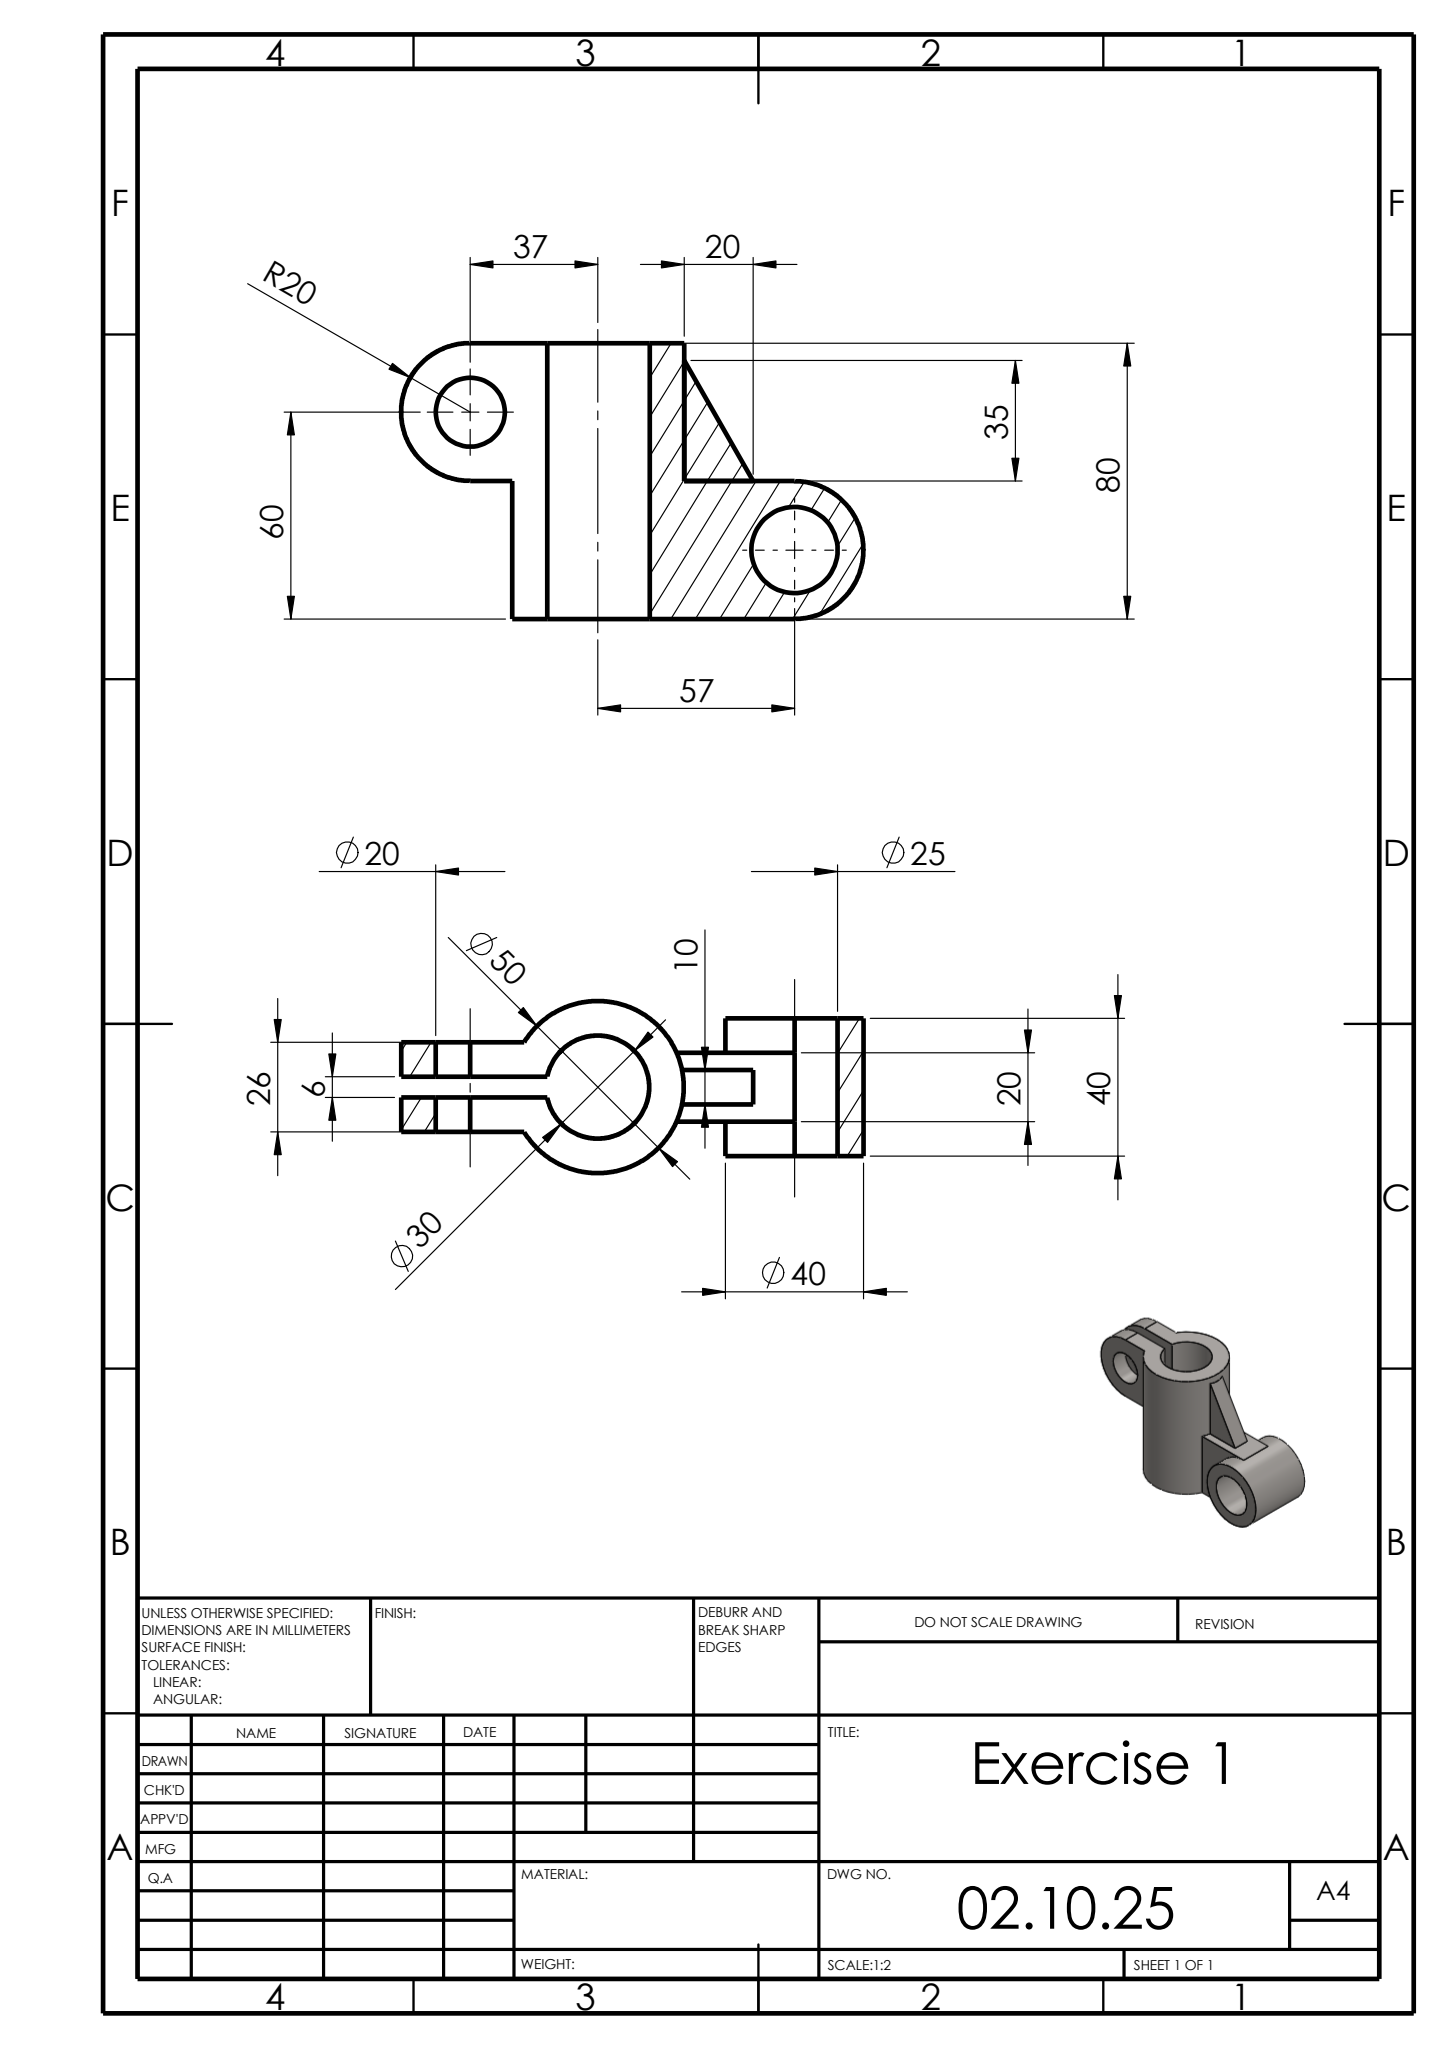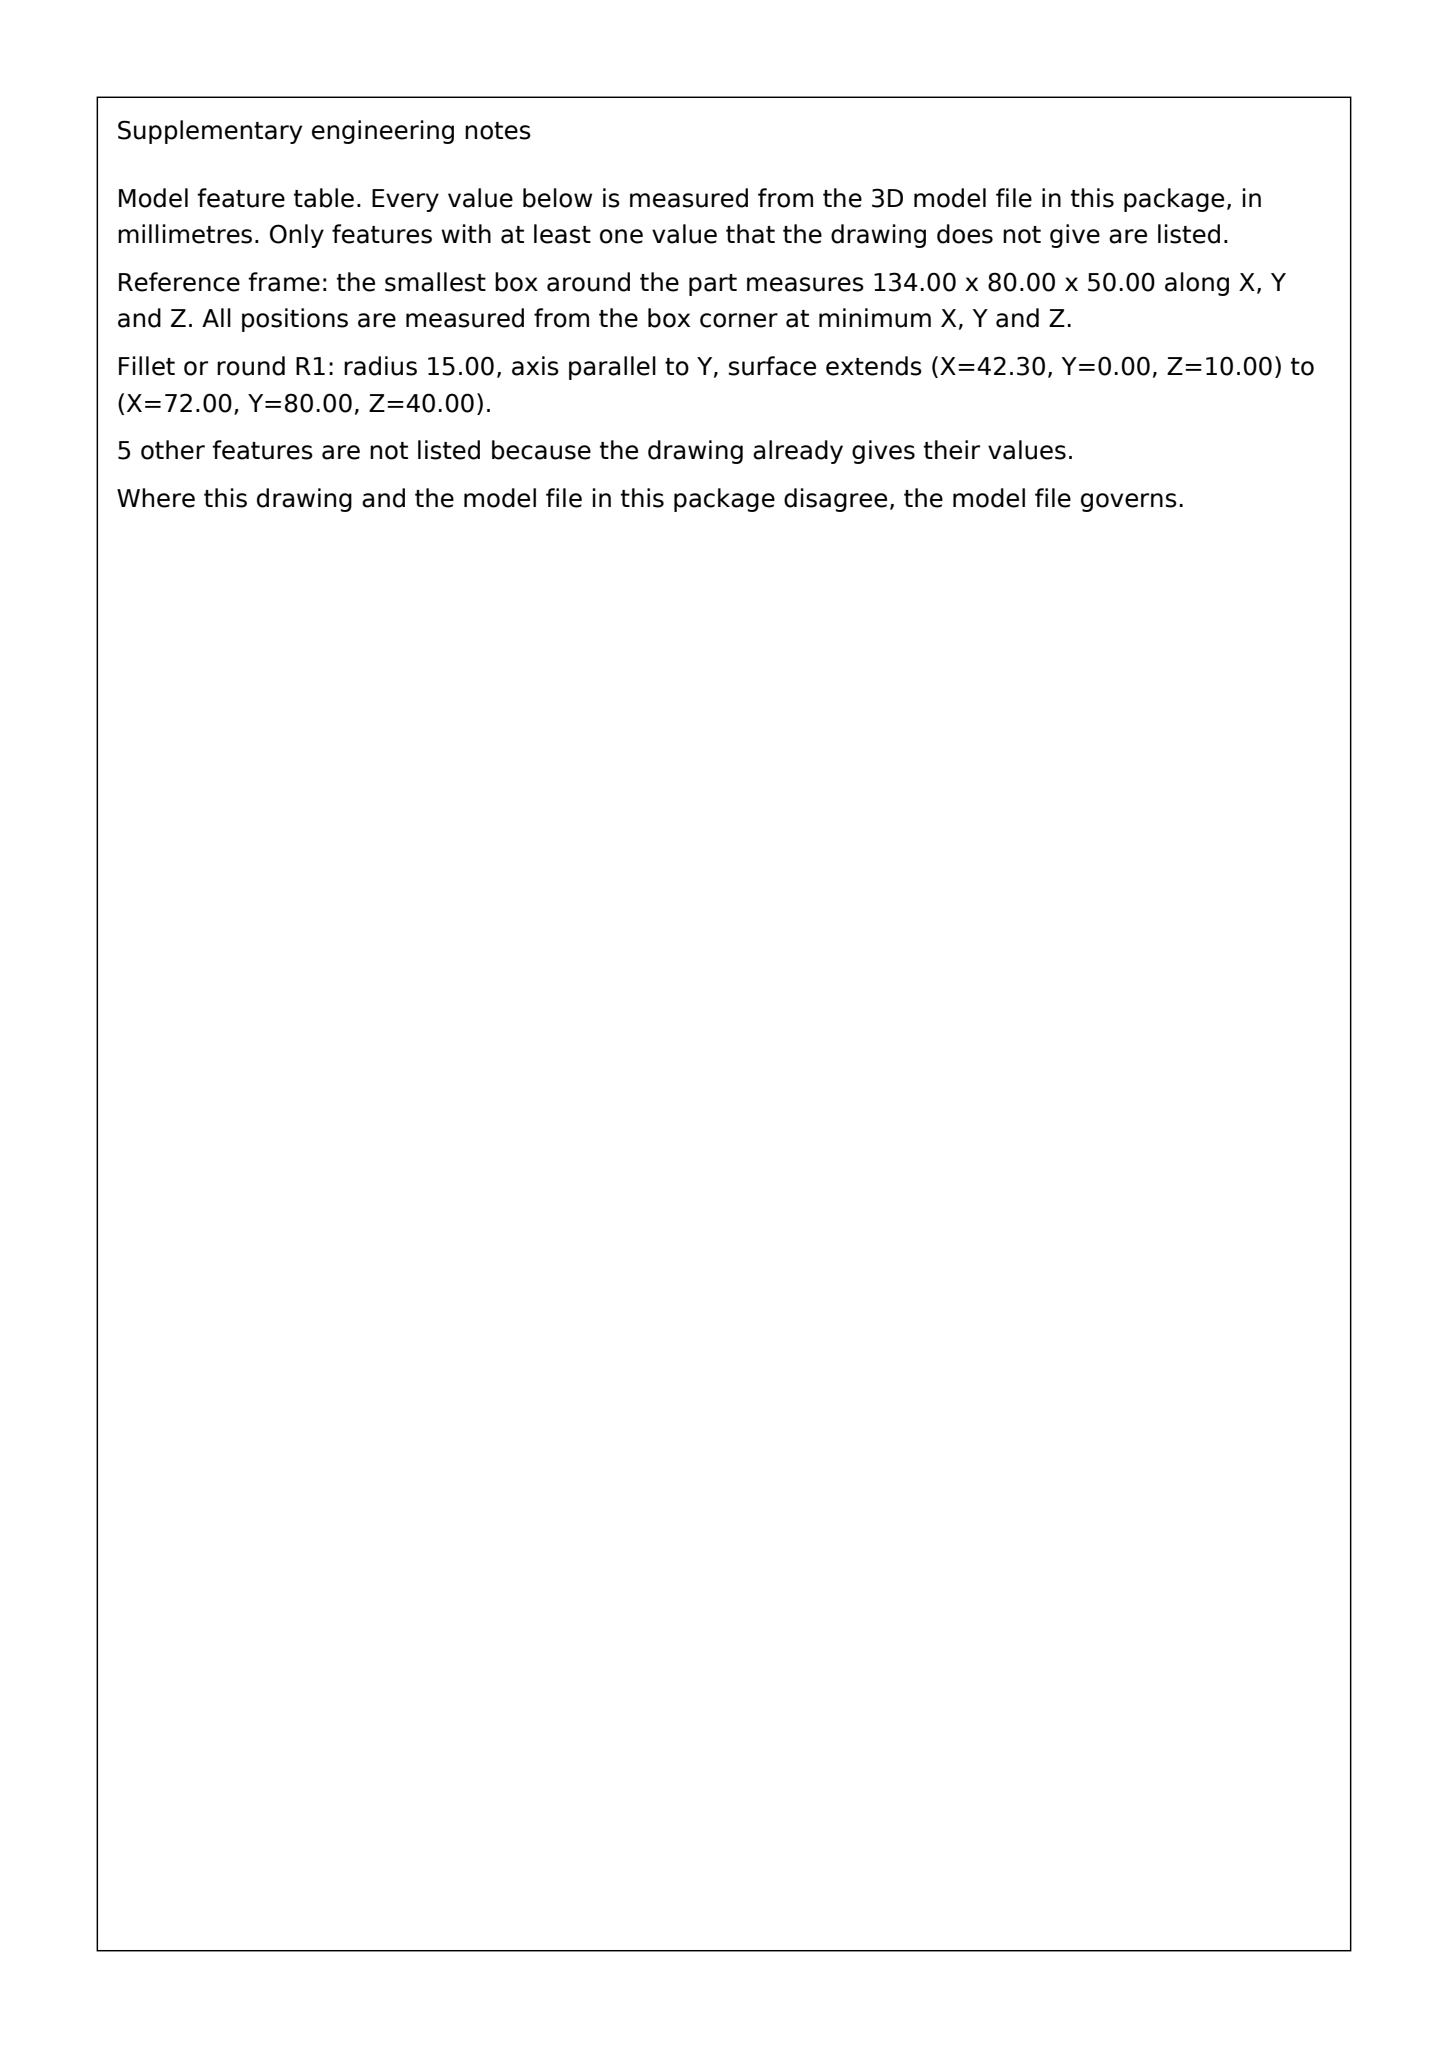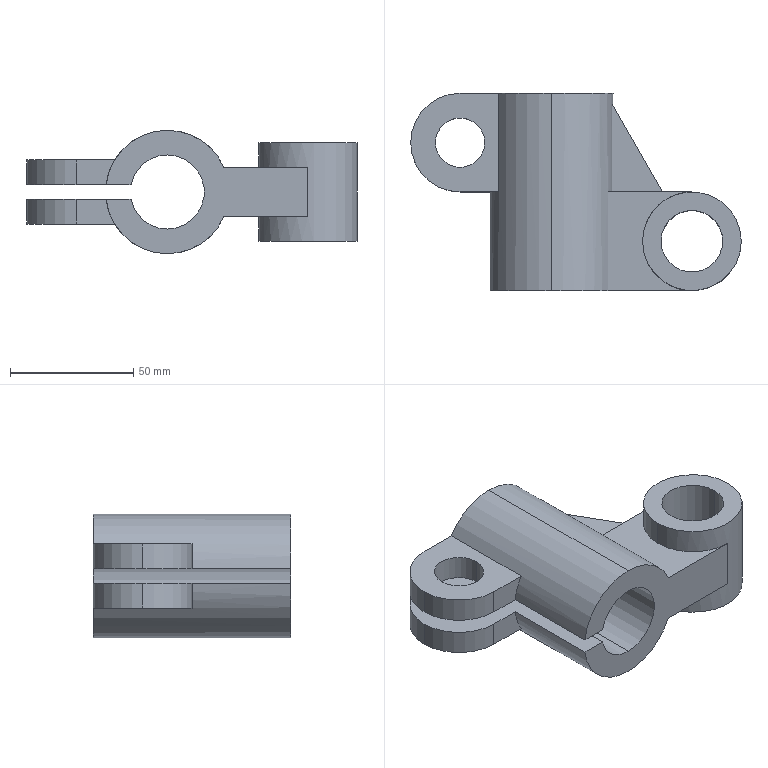Part | SolidWorks | mm | 1 solid | 34 faces | box 134 x 80 x 50 mm | volume 160575 mm3 | cylinder 18 | plane 16 | commonest cylinder face diameters 40 x6 20 x4 30 x3 50 x3 25 x2